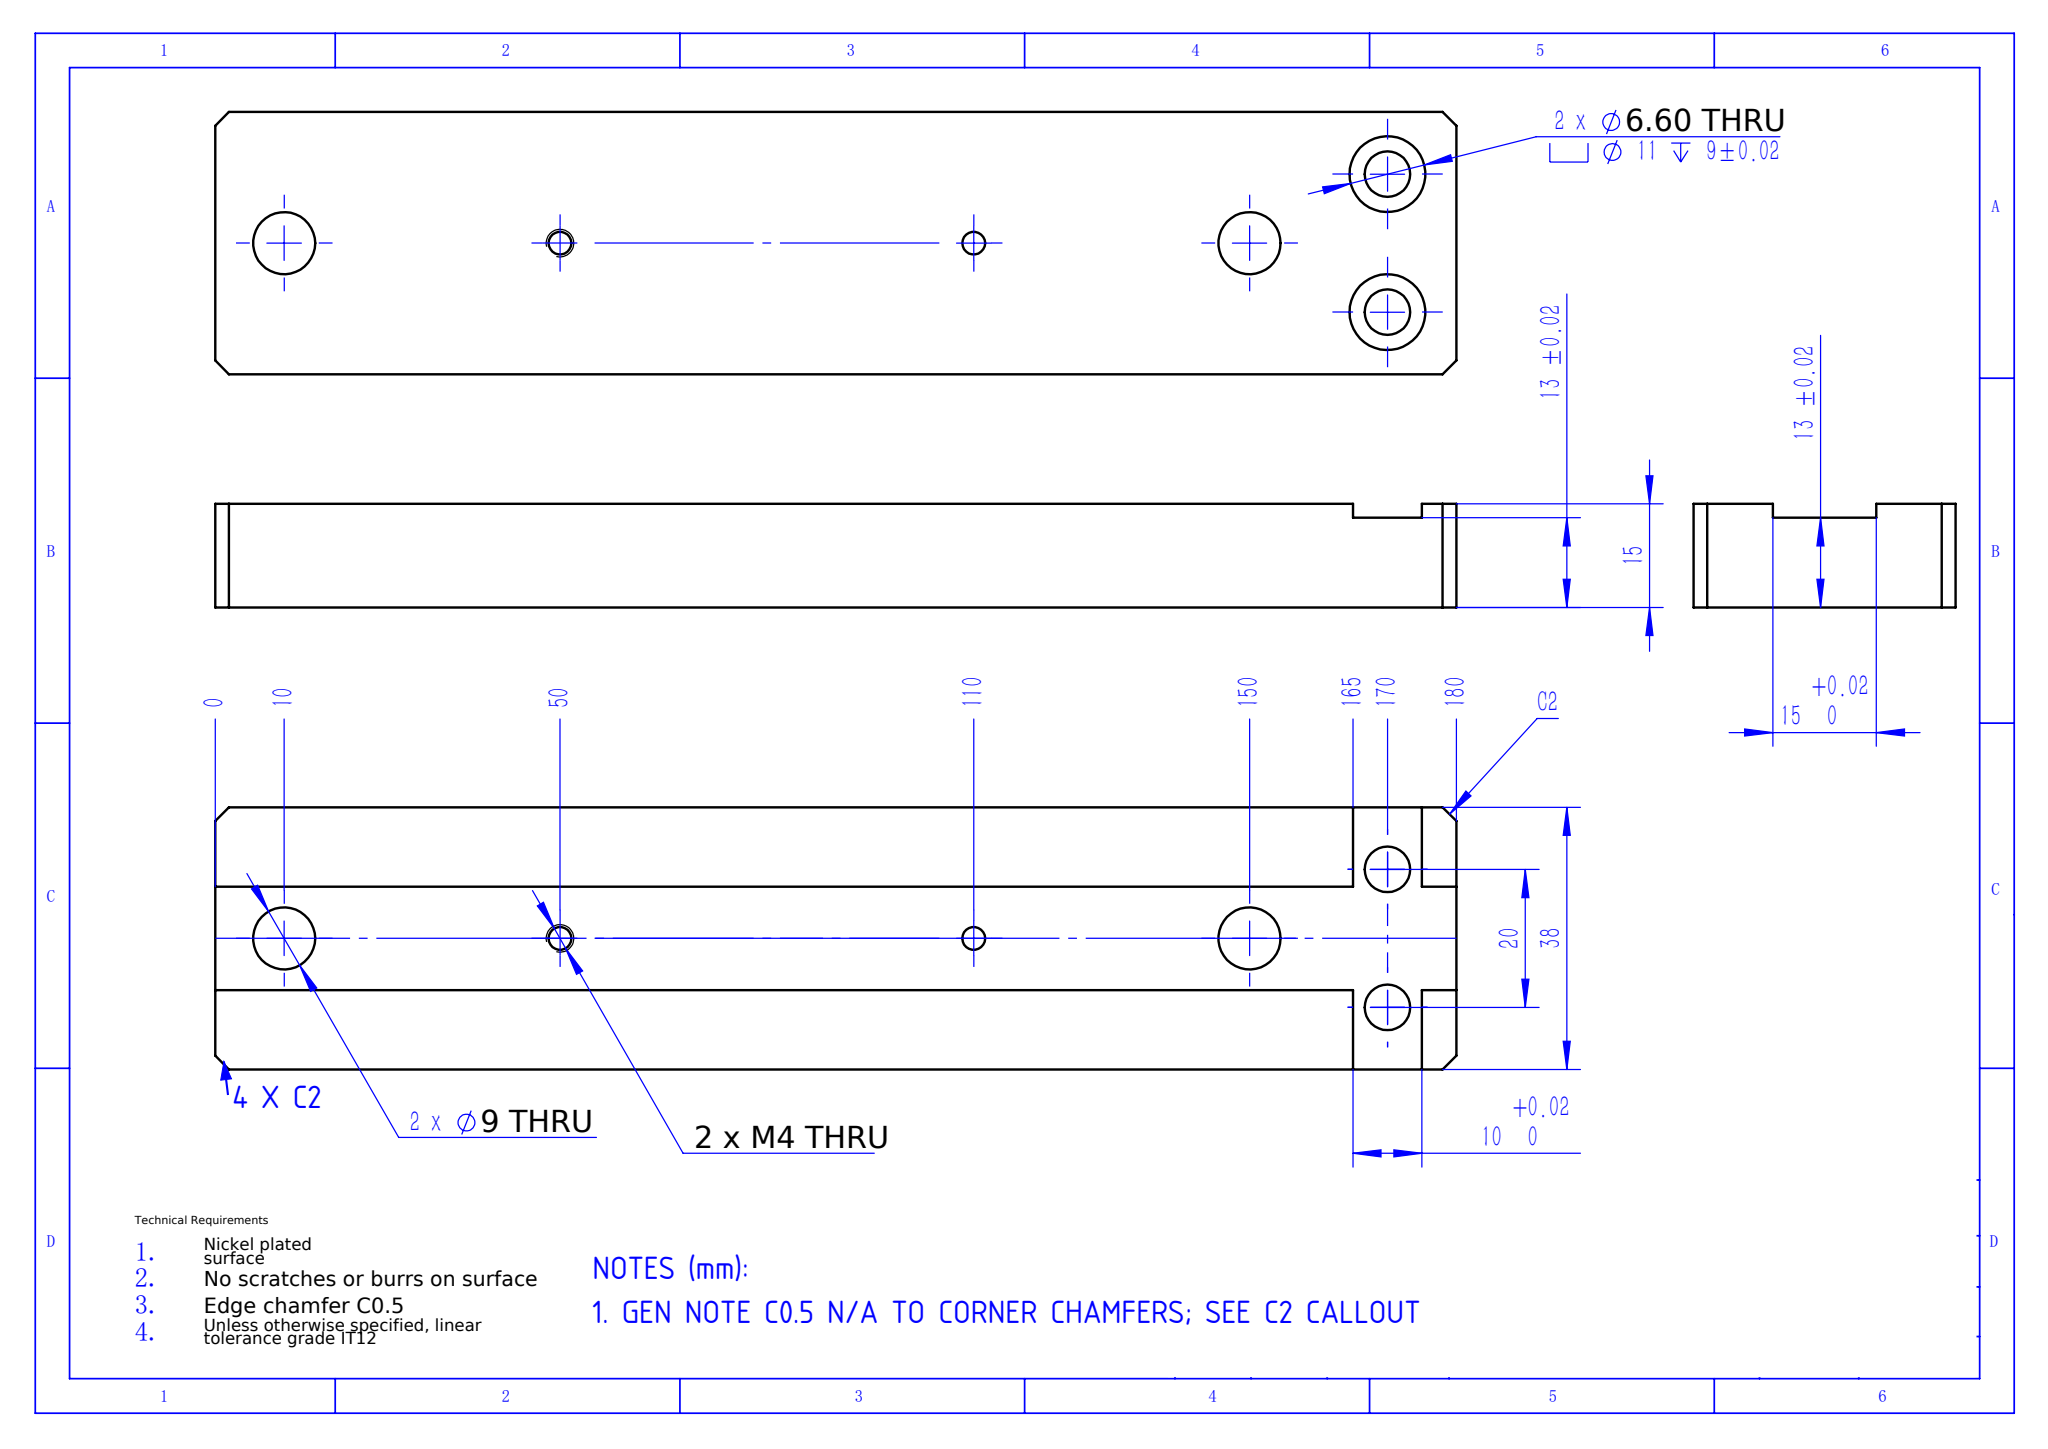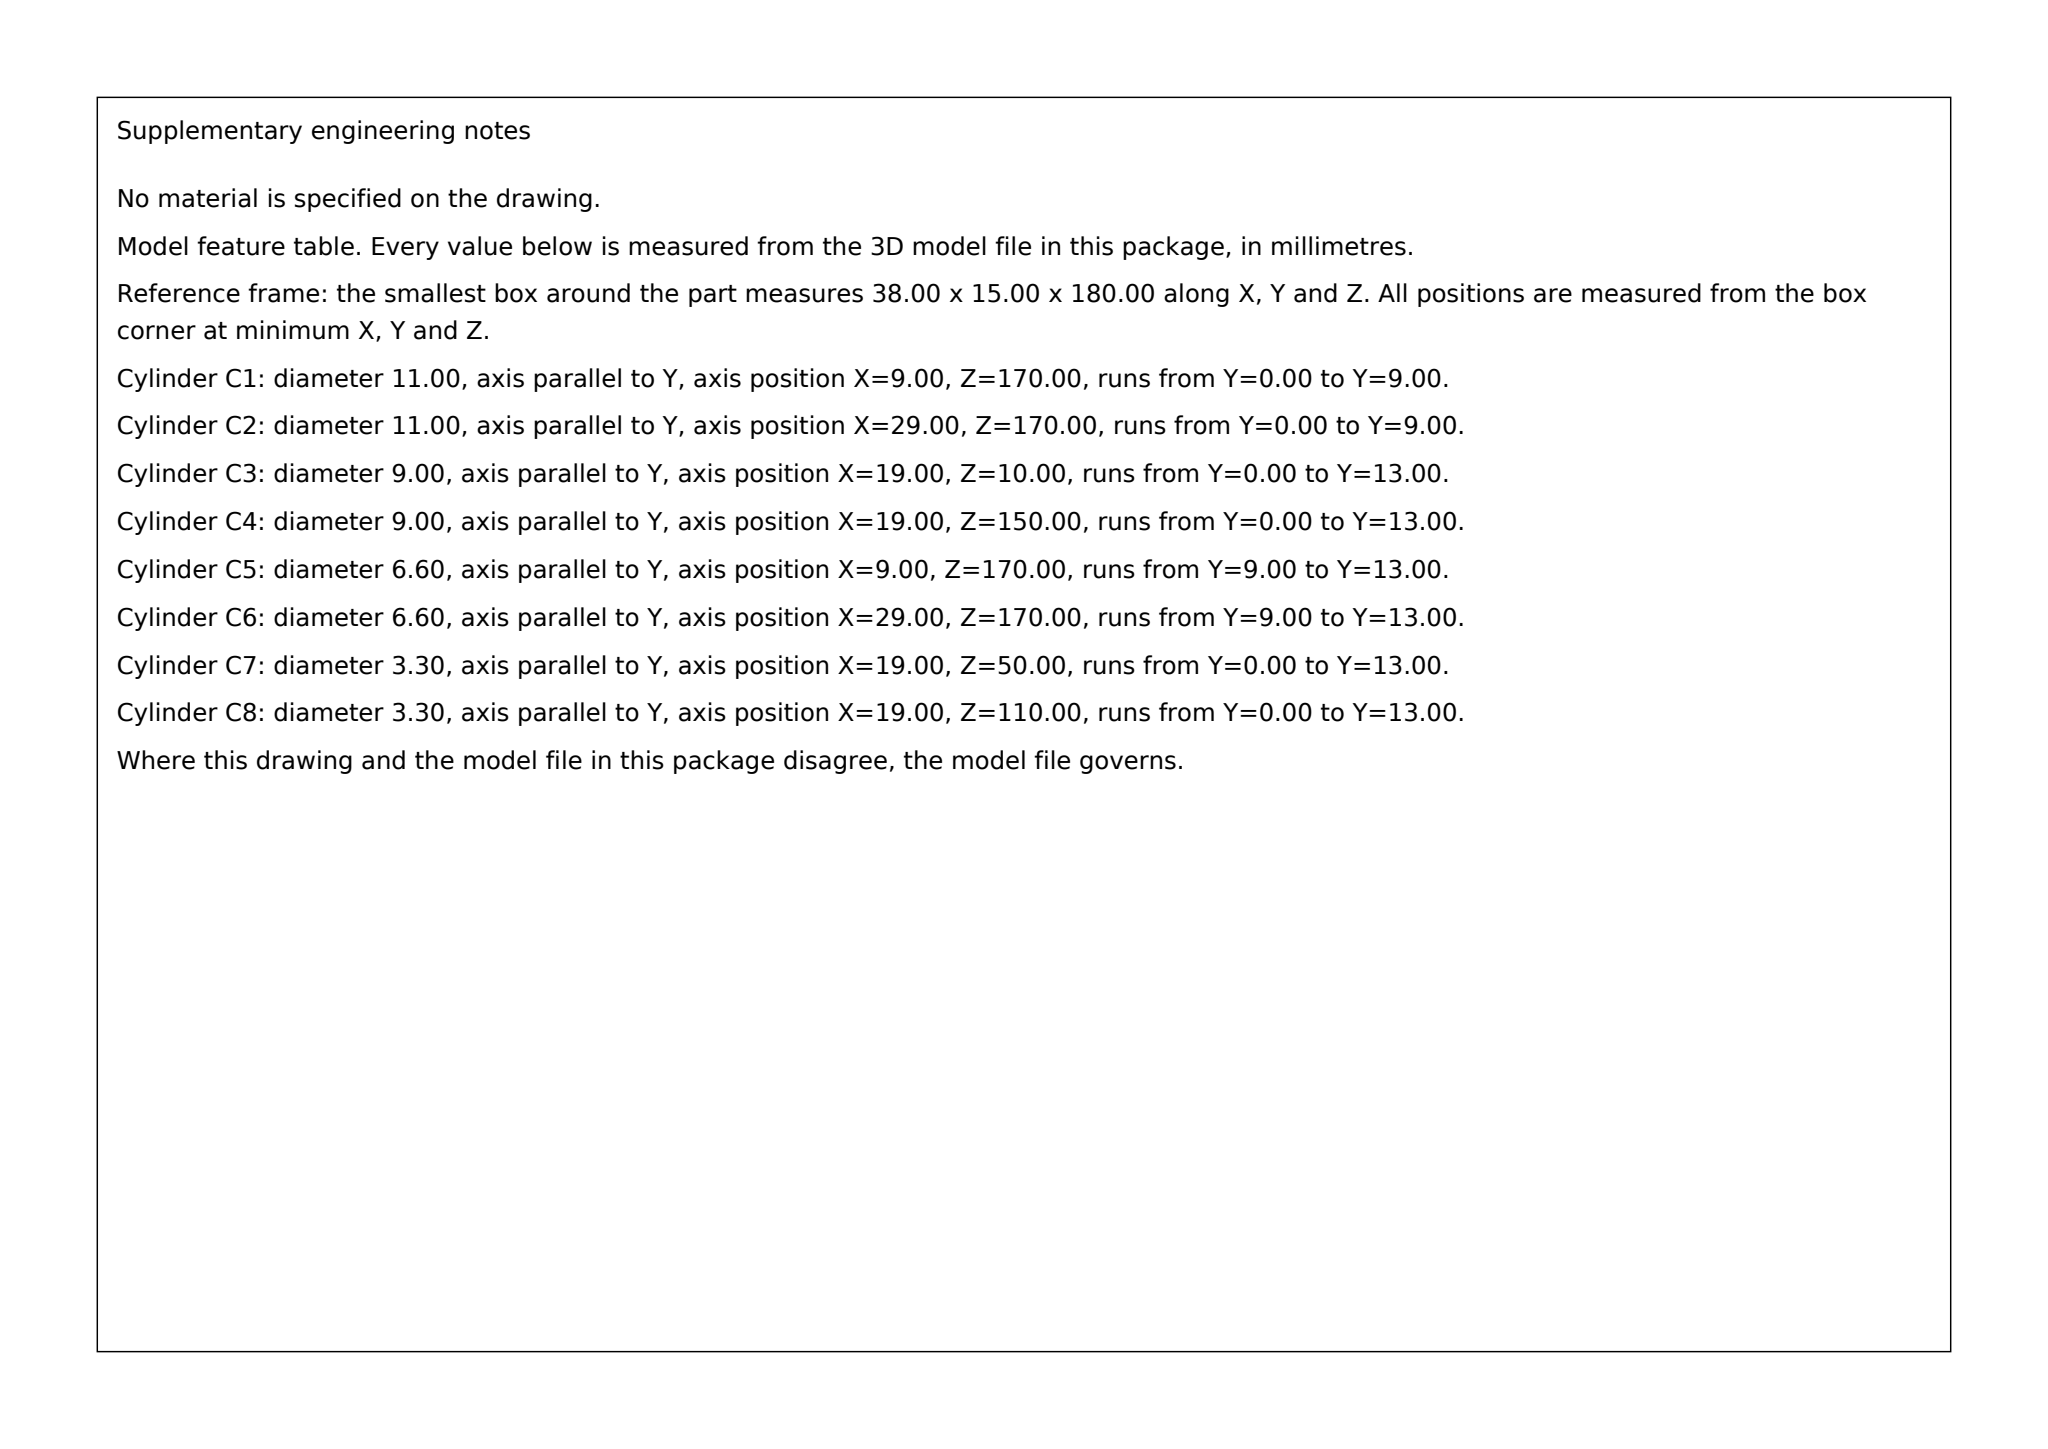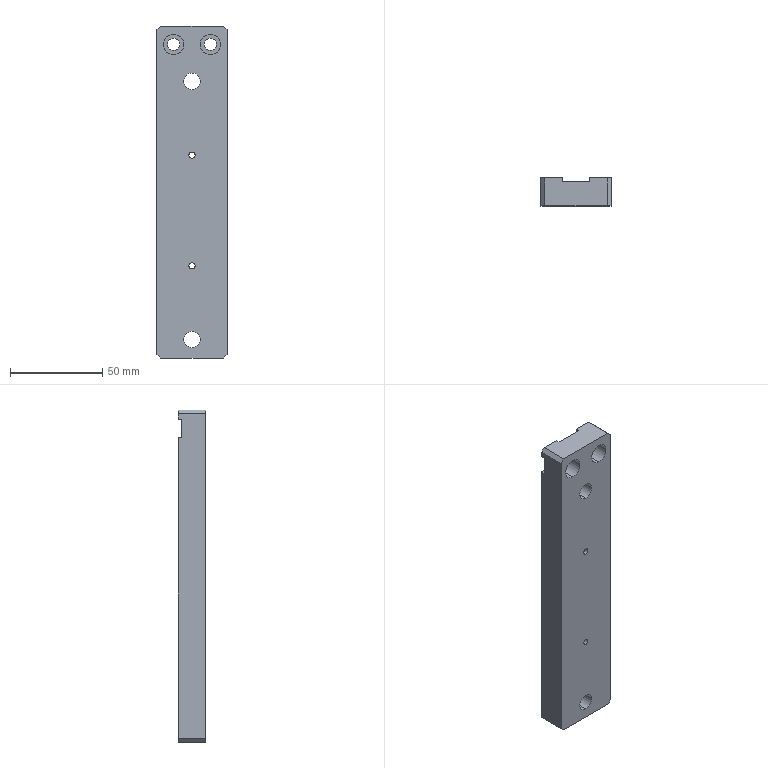Part | SolidWorks | mm | 1 solid | 40 faces | box 38 x 15 x 180 mm | volume 92759 mm3 | plane 24 | cylinder 16 | commonest cylinder face diameters 9 x4 11 x4 6.6 x4 3.3 x4
Drawing notes:
4 X C2 AT PLAN-VIEW CORNERS: 2 EA AT Z=0 AND Z=180 ENDS | from the solid: Bbox 38x15x180; corner chamfer faces at both z=0 and z=180 ends are non-axis-aligned (absent from axis_planes list x=0/38, z=0/180); no fillet_radii, no cones
GEN NOTE C0.5 N/A TO CORNER CHAMFERS; SEE C2 CALLOUT | from the solid: Chamfer faces at both ends are equal size, larger than 0.5; only axis planes x=0,38 / z=0,180 bound bbox
build123d program:
from build123d import *

# Parameters (mm, degrees)
SKETCH1_W                                         = 38
SKETCH1_H                                         = 180
BOSS_EXTRUDE1_DEPTH                               = 15
SKETCH2_W                                         = 15
SKETCH2_H                                         = 180
CUT_EXTRUDE1_DEPTH                                = 2
SKETCH3_W                                         = 38
SKETCH3_H                                         = 10
CUT_EXTRUDE2_DEPTH                                = 2
M4_TAPPED_HOLE1_D                                 = 3.3
LPATTERN1_COUNT                                   = 2
LPATTERN1_PITCH                                   = 60
HOLE_SIZE_ACCORDING_TO_HEXAGON_SOCKET_D           = 6.6
HOLE_SIZE_ACCORDING_TO_HEXAGON_SOCKET_CBORE_D     = 11
HOLE_SIZE_ACCORDING_TO_HEXAGON_SOCKET_CBORE_DEPTH = 9
M8_CLEARANCE_HOLE_1_D                             = 9
CHAMFER1_SIZE                                     = 2


with BuildPart() as part:
    # Sketch1 → Boss-Extrude1 (new body)
    with BuildSketch(Plane(origin=(0, 0, 0), x_dir=(1, 0, 0), z_dir=(0, 1, 0))):
        Rectangle(SKETCH1_W, SKETCH1_H)
    extrude(amount=BOSS_EXTRUDE1_DEPTH)

    # Sketch2 → Cut-Extrude1 (cut)
    with BuildSketch(Plane(origin=(0, 15, 0), x_dir=(1, 0, 0), z_dir=(0, 1, 0))):
        Rectangle(SKETCH2_W, SKETCH2_H)
    extrude(amount=-CUT_EXTRUDE1_DEPTH, mode=Mode.SUBTRACT)

    # Sketch3 → Cut-Extrude2 (cut)
    with BuildSketch(Plane(origin=(0, 15, 0), x_dir=(1, 0, 0), z_dir=(0, 1, 0))):
        with Locations((0, -80)):
            Rectangle(SKETCH3_W, SKETCH3_H)
    extrude(amount=-CUT_EXTRUDE2_DEPTH, mode=Mode.SUBTRACT)

    # M4 Tapped Hole1 (through all)
    with Locations(Plane(origin=(0, 15, 0), x_dir=(1, 0, 0), z_dir=(0, 1, 0))):
        with Locations((0, 40)):
            m4_tapped_hole1 = Hole(M4_TAPPED_HOLE1_D / 2)

    # LPattern1: M4 Tapped Hole1 ×2
    with Locations(*[(0, 0, i * LPATTERN1_PITCH) for i in range(1, LPATTERN1_COUNT)]):
        add(m4_tapped_hole1, mode=Mode.SUBTRACT)

    # Hole Size _ according to_ Hexagon Socket (through all)
    with Locations(Plane.XZ):
        with Locations((-10, 80), (10, 80)):
            CounterBoreHole(HOLE_SIZE_ACCORDING_TO_HEXAGON_SOCKET_D / 2, HOLE_SIZE_ACCORDING_TO_HEXAGON_SOCKET_CBORE_D / 2, HOLE_SIZE_ACCORDING_TO_HEXAGON_SOCKET_CBORE_DEPTH)

    # M8 Clearance Hole 1 (through all)
    with Locations(Plane(origin=(0, 13, 0), x_dir=(1, 0, 0), z_dir=(0, 1, 0))):
        with Locations((0, 80), (0, -60)):
            Hole(M8_CLEARANCE_HOLE_1_D / 2)

    # Chamfer1
    chamfer1_edges = [part.edges().sort_by_distance(p)[0] for p in [
        (19, 7.5, 90),
        (-19, 7.5, 90),
        (-19, 7.5, -90),
        (19, 7.5, -90),
    ]]
    chamfer(chamfer1_edges, length=CHAMFER1_SIZE)


solid = part.part